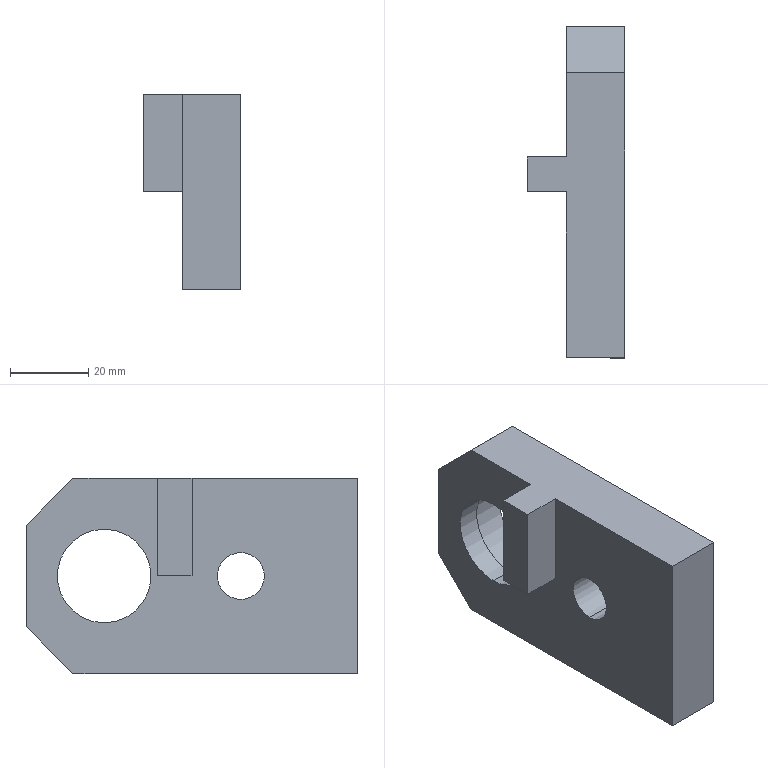Component | SolidWorks | BracketThree-1 | 1 solid | 19 faces | box 25 x 85 x 50 mm | volume 54632 mm3 | plane 13 | cylinder 6 | commonest cylinder face diameters 24 x2 26 x2 12 x2
build123d program:
from build123d import *

# Parameters (mm, degrees)
SKETCH1_R           = 6
BOSS_EXTRUDE1_DEPTH = 15
SKETCH2_R           = 13
CUT_EXTRUDE1_DEPTH  = 9
CUT_EXTRUDE2_REACH  = 52.122
SKETCH3_R           = 12
SKETCH4_W           = 25
SKETCH4_H           = 8.926
BOSS_EXTRUDE2_DEPTH = 10


with BuildPart() as part:
    # Sketch1 → Boss-Extrude1 (new body)
    with BuildSketch(Plane.XY):
        Polygon((-25, 30.5), (-13, 42.5), (13, 42.5), (25, 30.5), (25, -42.5), (-25, -42.5), align=None)
        with Locations((0, -12.5)):
            Circle(SKETCH1_R, mode=Mode.SUBTRACT)
    extrude(amount=BOSS_EXTRUDE1_DEPTH)

    # Sketch2 → Cut-Extrude1 (cut)
    with BuildSketch(Plane.XY.offset(15)):
        with Locations((0, 22.5)):
            Circle(SKETCH2_R)
    extrude(amount=-CUT_EXTRUDE1_DEPTH, mode=Mode.SUBTRACT)

    # Sketch3 → Cut-Extrude2 (cut, up to next)
    with BuildSketch(Plane.XY.offset(6), mode=Mode.PRIVATE) as cut_extrude2_sk1:
        with Locations((0, 22.5)):
            Circle(SKETCH3_R)
    cut_extrude2_tool1 = extrude(cut_extrude2_sk1.sketch, amount=-CUT_EXTRUDE2_REACH, mode=Mode.PRIVATE) & part.part
    add(cut_extrude2_tool1.solids().sort_by_distance((0, 22.5, 6))[0], mode=Mode.SUBTRACT)

    # Sketch4 → Boss-Extrude2 (add)
    with BuildSketch(Plane(origin=(0, 0, 0), x_dir=(-1, 0, 0), z_dir=(0, 0, -1))):
        with Locations((12.5, 4.463)):
            Rectangle(SKETCH4_W, SKETCH4_H)
    extrude(amount=BOSS_EXTRUDE2_DEPTH)


solid = part.part

# Placed as in the assembly
solid = solid.moved(Location((78.546, 54.5, 438.671), (0, 90, 0)))
STEP:
#1=CARTESIAN_POINT('',(3.092,3.031,16.798));
#2=VERTEX_POINT('',#1);
#3=CARTESIAN_POINT('',(3.092,3.031,17.743));
#4=VERTEX_POINT('',#3);
#5=CARTESIAN_POINT('',(3.092,3.031,17.271));
#6=DIRECTION('',(-1.,-0.,0.));
#7=DIRECTION('',(-0.,0.,-1.));
#8=AXIS2_PLACEMENT_3D('',#5,#6,#7);
#9=CIRCLE('',#8,0.4724);
#10=EDGE_CURVE('',#2,#4,#9,.T.);
#11=ORIENTED_EDGE('',*,*,#10,.T.);
#12=CARTESIAN_POINT('',(3.329,3.031,17.743));
#13=VERTEX_POINT('',#12);
#14=CARTESIAN_POINT('',(3.092,3.031,17.743));
#15=DIRECTION('',(1.,0.,-0.));
#16=VECTOR('',#15,39.37);
#17=LINE('',#14,#16);
#18=EDGE_CURVE('',#4,#13,#17,.T.);
#19=ORIENTED_EDGE('',*,*,#18,.T.);
#20=CARTESIAN_POINT('',(3.329,3.031,16.798));
#21=VERTEX_POINT('',#20);
#22=CARTESIAN_POINT('',(3.329,3.031,17.271));
#23=DIRECTION('',(1.,0.,-0.));
#24=DIRECTION('',(-0.,0.,-1.));
#25=AXIS2_PLACEMENT_3D('',#22,#23,#24);
#26=CIRCLE('',#25,0.4724);
#27=EDGE_CURVE('',#13,#21,#26,.T.);
#28=ORIENTED_EDGE('',*,*,#27,.T.);
#29=CARTESIAN_POINT('',(3.092,3.031,16.798));
#30=DIRECTION('',(1.,0.,-0.));
#31=VECTOR('',#30,39.37);
#32=LINE('',#29,#31);
#33=EDGE_CURVE('',#2,#21,#32,.T.);
#34=ORIENTED_EDGE('',*,*,#33,.F.);
#35=EDGE_LOOP('',(#11,#19,#28,#34));
#36=FACE_OUTER_BOUND('',#35,.T.);
#37=CARTESIAN_POINT('',(3.092,3.031,17.271));
#38=DIRECTION('',(1.,0.,-0.));
#39=DIRECTION('',(-0.,0.,-1.));
#40=AXIS2_PLACEMENT_3D('',#37,#38,#39);
#41=CYLINDRICAL_SURFACE('',#40,0.4724);
#42=ADVANCED_FACE('',(#36),#41,.F.);
#43=CARTESIAN_POINT('',(3.329,3.031,17.782));
#44=VERTEX_POINT('',#43);
#45=CARTESIAN_POINT('',(3.329,3.031,16.759));
#46=VERTEX_POINT('',#45);
#47=CARTESIAN_POINT('',(3.329,3.031,17.271));
#48=DIRECTION('',(1.,0.,-0.));
#49=DIRECTION('',(-0.,0.,-1.));
#50=AXIS2_PLACEMENT_3D('',#47,#48,#49);
#51=CIRCLE('',#50,0.5118);
#52=EDGE_CURVE('',#44,#46,#51,.T.);
#53=ORIENTED_EDGE('',*,*,#52,.F.);
#54=CARTESIAN_POINT('',(3.683,3.031,17.782));
#55=VERTEX_POINT('',#54);
#56=CARTESIAN_POINT('',(3.329,3.031,17.782));
#57=DIRECTION('',(1.,0.,-0.));
#58=VECTOR('',#57,39.37);
#59=LINE('',#56,#58);
#60=EDGE_CURVE('',#44,#55,#59,.T.);
#61=ORIENTED_EDGE('',*,*,#60,.T.);
#62=CARTESIAN_POINT('',(3.683,3.031,16.759));
#63=VERTEX_POINT('',#62);
#64=CARTESIAN_POINT('',(3.683,3.031,17.271));
#65=DIRECTION('',(1.,0.,-0.));
#66=DIRECTION('',(-0.,0.,-1.));
#67=AXIS2_PLACEMENT_3D('',#64,#65,#66);
#68=CIRCLE('',#67,0.5118);
#69=EDGE_CURVE('',#55,#63,#68,.T.);
#70=ORIENTED_EDGE('',*,*,#69,.T.);
#71=CARTESIAN_POINT('',(3.329,3.031,16.759));
#72=DIRECTION('',(1.,0.,-0.));
#73=VECTOR('',#72,39.37);
#74=LINE('',#71,#73);
#75=EDGE_CURVE('',#46,#63,#74,.T.);
#76=ORIENTED_EDGE('',*,*,#75,.F.);
#77=EDGE_LOOP('',(#53,#61,#70,#76));
#78=FACE_OUTER_BOUND('',#77,.T.);
#79=CARTESIAN_POINT('',(3.329,3.031,17.271));
#80=DIRECTION('',(1.,0.,-0.));
#81=DIRECTION('',(-0.,0.,-1.));
#82=AXIS2_PLACEMENT_3D('',#79,#80,#81);
#83=CYLINDRICAL_SURFACE('',#82,0.5118);
#84=ADVANCED_FACE('',(#78),#83,.F.);
#85=CARTESIAN_POINT('',(3.683,1.654,17.507));
#86=VERTEX_POINT('',#85);
#87=CARTESIAN_POINT('',(3.683,1.654,17.034));
#88=VERTEX_POINT('',#87);
#89=CARTESIAN_POINT('',(3.683,1.654,17.271));
#90=DIRECTION('',(1.,0.,-0.));
#91=DIRECTION('',(-0.,0.,-1.));
#92=AXIS2_PLACEMENT_3D('',#89,#90,#91);
#93=CIRCLE('',#92,0.2362);
#94=EDGE_CURVE('',#86,#88,#93,.T.);
#95=ORIENTED_EDGE('',*,*,#94,.T.);
#96=CARTESIAN_POINT('',(3.092,1.654,17.034));
#97=VERTEX_POINT('',#96);
#98=CARTESIAN_POINT('',(3.683,1.654,17.034));
#99=DIRECTION('',(-1.,-0.,0.));
#100=VECTOR('',#99,39.37);
#101=LINE('',#98,#100);
#102=EDGE_CURVE('',#88,#97,#101,.T.);
#103=ORIENTED_EDGE('',*,*,#102,.T.);
#104=CARTESIAN_POINT('',(3.092,1.654,17.507));
#105=VERTEX_POINT('',#104);
#106=CARTESIAN_POINT('',(3.092,1.654,17.271));
#107=DIRECTION('',(1.,0.,-0.));
#108=DIRECTION('',(-0.,0.,-1.));
#109=AXIS2_PLACEMENT_3D('',#106,#107,#108);
#110=CIRCLE('',#109,0.2362);
#111=EDGE_CURVE('',#105,#97,#110,.T.);
#112=ORIENTED_EDGE('',*,*,#111,.F.);
#113=CARTESIAN_POINT('',(3.683,1.654,17.507));
#114=DIRECTION('',(-1.,-0.,0.));
#115=VECTOR('',#114,39.37);
#116=LINE('',#113,#115);
#117=EDGE_CURVE('',#86,#105,#116,.T.);
#118=ORIENTED_EDGE('',*,*,#117,.F.);
#119=EDGE_LOOP('',(#95,#103,#112,#118));
#120=FACE_OUTER_BOUND('',#119,.T.);
#121=CARTESIAN_POINT('',(3.683,1.654,17.271));
#122=DIRECTION('',(-1.,-0.,0.));
#123=DIRECTION('',(0.,0.,1.));
#124=AXIS2_PLACEMENT_3D('',#121,#122,#123);
#125=CYLINDRICAL_SURFACE('',#124,0.2362);
#126=ADVANCED_FACE('',(#120),#125,.F.);
#127=ORIENTED_EDGE('',*,*,#111,.T.);
#128=CARTESIAN_POINT('',(3.092,1.654,17.271));
#129=DIRECTION('',(1.,0.,-0.));
#130=DIRECTION('',(-0.,0.,-1.));
#131=AXIS2_PLACEMENT_3D('',#128,#129,#130);
#132=CIRCLE('',#131,0.2362);
#133=EDGE_CURVE('',#97,#105,#132,.T.);
#134=ORIENTED_EDGE('',*,*,#133,.T.);
#135=EDGE_LOOP('',(#127,#134));
#136=FACE_BOUND('',#135,.T.);
#137=ORIENTED_EDGE('',*,*,#10,.F.);
#138=CARTESIAN_POINT('',(3.092,3.031,17.271));
#139=DIRECTION('',(-1.,-0.,0.));
#140=DIRECTION('',(-0.,0.,-1.));
#141=AXIS2_PLACEMENT_3D('',#138,#139,#140);
#142=CIRCLE('',#141,0.4724);
#143=EDGE_CURVE('',#4,#2,#142,.T.);
#144=ORIENTED_EDGE('',*,*,#143,.F.);
#145=EDGE_LOOP('',(#137,#144));
#146=FACE_BOUND('',#145,.T.);
#147=CARTESIAN_POINT('',(3.092,2.497,18.255));
#148=VERTEX_POINT('',#147);
#149=CARTESIAN_POINT('',(3.092,2.497,17.271));
#150=VERTEX_POINT('',#149);
#151=CARTESIAN_POINT('',(3.092,2.497,17.271));
#152=DIRECTION('',(-0.,-0.,-1.));
#153=VECTOR('',#152,39.37);
#154=LINE('',#151,#153);
#155=EDGE_CURVE('',#148,#150,#154,.T.);
#156=ORIENTED_EDGE('',*,*,#155,.F.);
#157=CARTESIAN_POINT('',(3.092,3.346,18.255));
#158=VERTEX_POINT('',#157);
#159=CARTESIAN_POINT('',(3.092,3.346,18.255));
#160=DIRECTION('',(0.,-1.,-0.));
#161=VECTOR('',#160,39.37);
#162=LINE('',#159,#161);
#163=EDGE_CURVE('',#158,#148,#162,.T.);
#164=ORIENTED_EDGE('',*,*,#163,.F.);
#165=CARTESIAN_POINT('',(3.092,3.819,17.782));
#166=VERTEX_POINT('',#165);
#167=CARTESIAN_POINT('',(3.092,3.346,18.255));
#168=DIRECTION('',(0.,-0.7071,0.7071));
#169=VECTOR('',#168,39.37);
#170=LINE('',#167,#169);
#171=EDGE_CURVE('',#166,#158,#170,.T.);
#172=ORIENTED_EDGE('',*,*,#171,.F.);
#173=CARTESIAN_POINT('',(3.092,3.819,16.759));
#174=VERTEX_POINT('',#173);
#175=CARTESIAN_POINT('',(3.092,3.819,17.782));
#176=DIRECTION('',(0.,0.,1.));
#177=VECTOR('',#176,39.37);
#178=LINE('',#175,#177);
#179=EDGE_CURVE('',#174,#166,#178,.T.);
#180=ORIENTED_EDGE('',*,*,#179,.F.);
#181=CARTESIAN_POINT('',(3.092,3.346,16.286));
#182=VERTEX_POINT('',#181);
#183=CARTESIAN_POINT('',(3.092,3.819,16.759));
#184=DIRECTION('',(0.,0.7071,0.7071));
#185=VECTOR('',#184,39.37);
#186=LINE('',#183,#185);
#187=EDGE_CURVE('',#182,#174,#186,.T.);
#188=ORIENTED_EDGE('',*,*,#187,.F.);
#189=CARTESIAN_POINT('',(3.092,0.4724,16.286));
#190=VERTEX_POINT('',#189);
#191=CARTESIAN_POINT('',(3.092,3.346,16.286));
#192=DIRECTION('',(-0.,1.,-0.));
#193=VECTOR('',#192,39.37);
#194=LINE('',#191,#193);
#195=EDGE_CURVE('',#190,#182,#194,.T.);
#196=ORIENTED_EDGE('',*,*,#195,.F.);
#197=CARTESIAN_POINT('',(3.092,0.4724,18.255));
#198=VERTEX_POINT('',#197);
#199=CARTESIAN_POINT('',(3.092,0.4724,18.255));
#200=DIRECTION('',(-0.,-0.,-1.));
#201=VECTOR('',#200,39.37);
#202=LINE('',#199,#201);
#203=EDGE_CURVE('',#198,#190,#202,.T.);
#204=ORIENTED_EDGE('',*,*,#203,.F.);
#205=CARTESIAN_POINT('',(3.092,2.146,18.255));
#206=VERTEX_POINT('',#205);
#207=CARTESIAN_POINT('',(3.092,3.346,18.255));
#208=DIRECTION('',(0.,-1.,-0.));
#209=VECTOR('',#208,39.37);
#210=LINE('',#207,#209);
#211=EDGE_CURVE('',#206,#198,#210,.T.);
#212=ORIENTED_EDGE('',*,*,#211,.F.);
#213=CARTESIAN_POINT('',(3.092,2.146,17.271));
#214=VERTEX_POINT('',#213);
#215=CARTESIAN_POINT('',(3.092,2.146,17.271));
#216=DIRECTION('',(0.,0.,1.));
#217=VECTOR('',#216,39.37);
#218=LINE('',#215,#217);
#219=EDGE_CURVE('',#214,#206,#218,.T.);
#220=ORIENTED_EDGE('',*,*,#219,.F.);
#221=CARTESIAN_POINT('',(3.092,2.146,17.271));
#222=DIRECTION('',(0.,-1.,0.));
#223=VECTOR('',#222,39.37);
#224=LINE('',#221,#223);
#225=EDGE_CURVE('',#150,#214,#224,.T.);
#226=ORIENTED_EDGE('',*,*,#225,.F.);
#227=EDGE_LOOP('',(#156,#164,#172,#180,#188,#196,#204,#212,#220,#226));
#228=FACE_OUTER_BOUND('',#227,.T.);
#229=CARTESIAN_POINT('',(3.092,2.146,17.271));
#230=DIRECTION('',(1.,0.,-0.));
#231=DIRECTION('',(-0.,-0.,-1.));
#232=AXIS2_PLACEMENT_3D('',#229,#230,#231);
#233=PLANE('',#232);
#234=ADVANCED_FACE('',(#136,#146,#228),#233,.F.);
#235=CARTESIAN_POINT('',(3.683,3.031,17.271));
#236=DIRECTION('',(1.,0.,-0.));
#237=DIRECTION('',(-0.,0.,-1.));
#238=AXIS2_PLACEMENT_3D('',#235,#236,#237);
#239=CIRCLE('',#238,0.5118);
#240=EDGE_CURVE('',#63,#55,#239,.T.);
#241=ORIENTED_EDGE('',*,*,#240,.F.);
#242=ORIENTED_EDGE('',*,*,#69,.F.);
#243=EDGE_LOOP('',(#241,#242));
#244=FACE_BOUND('',#243,.T.);
#245=CARTESIAN_POINT('',(3.683,0.4724,16.286));
#246=VERTEX_POINT('',#245);
#247=CARTESIAN_POINT('',(3.683,3.346,16.286));
#248=VERTEX_POINT('',#247);
#249=CARTESIAN_POINT('',(3.683,3.346,16.286));
#250=DIRECTION('',(-0.,1.,-0.));
#251=VECTOR('',#250,39.37);
#252=LINE('',#249,#251);
#253=EDGE_CURVE('',#246,#248,#252,.T.);
#254=ORIENTED_EDGE('',*,*,#253,.T.);
#255=CARTESIAN_POINT('',(3.683,3.819,16.759));
#256=VERTEX_POINT('',#255);
#257=CARTESIAN_POINT('',(3.683,3.819,16.759));
#258=DIRECTION('',(0.,0.7071,0.7071));
#259=VECTOR('',#258,39.37);
#260=LINE('',#257,#259);
#261=EDGE_CURVE('',#248,#256,#260,.T.);
#262=ORIENTED_EDGE('',*,*,#261,.T.);
#263=CARTESIAN_POINT('',(3.683,3.819,17.782));
#264=VERTEX_POINT('',#263);
#265=CARTESIAN_POINT('',(3.683,3.819,17.782));
#266=DIRECTION('',(0.,0.,1.));
#267=VECTOR('',#266,39.37);
#268=LINE('',#265,#267);
#269=EDGE_CURVE('',#256,#264,#268,.T.);
#270=ORIENTED_EDGE('',*,*,#269,.T.);
#271=CARTESIAN_POINT('',(3.683,3.346,18.255));
#272=VERTEX_POINT('',#271);
#273=CARTESIAN_POINT('',(3.683,3.346,18.255));
#274=DIRECTION('',(0.,-0.7071,0.7071));
#275=VECTOR('',#274,39.37);
#276=LINE('',#273,#275);
#277=EDGE_CURVE('',#264,#272,#276,.T.);
#278=ORIENTED_EDGE('',*,*,#277,.T.);
#279=CARTESIAN_POINT('',(3.683,0.4724,18.255));
#280=VERTEX_POINT('',#279);
#281=CARTESIAN_POINT('',(3.683,3.346,18.255));
#282=DIRECTION('',(0.,-1.,-0.));
#283=VECTOR('',#282,39.37);
#284=LINE('',#281,#283);
#285=EDGE_CURVE('',#272,#280,#284,.T.);
#286=ORIENTED_EDGE('',*,*,#285,.T.);
#287=CARTESIAN_POINT('',(3.683,0.4724,18.255));
#288=DIRECTION('',(-0.,-0.,-1.));
#289=VECTOR('',#288,39.37);
#290=LINE('',#287,#289);
#291=EDGE_CURVE('',#280,#246,#290,.T.);
#292=ORIENTED_EDGE('',*,*,#291,.T.);
#293=EDGE_LOOP('',(#254,#262,#270,#278,#286,#292));
#294=FACE_OUTER_BOUND('',#293,.T.);
#295=ORIENTED_EDGE('',*,*,#94,.F.);
#296=CARTESIAN_POINT('',(3.683,1.654,17.271));
#297=DIRECTION('',(1.,0.,-0.));
#298=DIRECTION('',(-0.,0.,-1.));
#299=AXIS2_PLACEMENT_3D('',#296,#297,#298);
#300=CIRCLE('',#299,0.2362);
#301=EDGE_CURVE('',#88,#86,#300,.T.);
#302=ORIENTED_EDGE('',*,*,#301,.F.);
#303=EDGE_LOOP('',(#295,#302));
#304=FACE_BOUND('',#303,.T.);
#305=CARTESIAN_POINT('',(3.683,2.146,17.271));
#306=DIRECTION('',(1.,0.,-0.));
#307=DIRECTION('',(-0.,-0.,-1.));
#308=AXIS2_PLACEMENT_3D('',#305,#306,#307);
#309=PLANE('',#308);
#310=ADVANCED_FACE('',(#244,#294,#304),#309,.T.);
#311=ORIENTED_EDGE('',*,*,#195,.T.);
#312=CARTESIAN_POINT('',(3.683,3.346,16.286));
#313=DIRECTION('',(-1.,-0.,0.));
#314=VECTOR('',#313,39.37);
#315=LINE('',#312,#314);
#316=EDGE_CURVE('',#248,#182,#315,.T.);
#317=ORIENTED_EDGE('',*,*,#316,.F.);
#318=ORIENTED_EDGE('',*,*,#253,.F.);
#319=CARTESIAN_POINT('',(3.683,0.4724,16.286));
#320=DIRECTION('',(-1.,-0.,0.));
#321=VECTOR('',#320,39.37);
#322=LINE('',#319,#321);
#323=EDGE_CURVE('',#246,#190,#322,.T.);
#324=ORIENTED_EDGE('',*,*,#323,.T.);
#325=EDGE_LOOP('',(#311,#317,#318,#324));
#326=FACE_OUTER_BOUND('',#325,.T.);
#327=CARTESIAN_POINT('',(3.683,3.346,16.286));
#328=DIRECTION('',(0.,0.,1.));
#329=DIRECTION('',(0.,-1.,0.));
#330=AXIS2_PLACEMENT_3D('',#327,#328,#329);
#331=PLANE('',#330);
#332=ADVANCED_FACE('',(#326),#331,.F.);
#333=ORIENTED_EDGE('',*,*,#187,.T.);
#334=CARTESIAN_POINT('',(3.683,3.819,16.759));
#335=DIRECTION('',(-1.,-0.,0.));
#336=VECTOR('',#335,39.37);
#337=LINE('',#334,#336);
#338=EDGE_CURVE('',#256,#174,#337,.T.);
#339=ORIENTED_EDGE('',*,*,#338,.F.);
#340=ORIENTED_EDGE('',*,*,#261,.F.);
#341=ORIENTED_EDGE('',*,*,#316,.T.);
#342=EDGE_LOOP('',(#333,#339,#340,#341));
#343=FACE_OUTER_BOUND('',#342,.T.);
#344=CARTESIAN_POINT('',(3.683,3.819,16.759));
#345=DIRECTION('',(0.,-0.7071,0.7071));
#346=DIRECTION('',(-0.,-0.7071,-0.7071));
#347=AXIS2_PLACEMENT_3D('',#344,#345,#346);
#348=PLANE('',#347);
#349=ADVANCED_FACE('',(#343),#348,.F.);
#350=ORIENTED_EDGE('',*,*,#179,.T.);
#351=CARTESIAN_POINT('',(3.683,3.819,17.782));
#352=DIRECTION('',(-1.,-0.,0.));
#353=VECTOR('',#352,39.37);
#354=LINE('',#351,#353);
#355=EDGE_CURVE('',#264,#166,#354,.T.);
#356=ORIENTED_EDGE('',*,*,#355,.F.);
#357=ORIENTED_EDGE('',*,*,#269,.F.);
#358=ORIENTED_EDGE('',*,*,#338,.T.);
#359=EDGE_LOOP('',(#350,#356,#357,#358));
#360=FACE_OUTER_BOUND('',#359,.T.);
#361=CARTESIAN_POINT('',(3.683,3.819,17.782));
#362=DIRECTION('',(0.,-1.,0.));
#363=DIRECTION('',(-1.,-0.,0.));
#364=AXIS2_PLACEMENT_3D('',#361,#362,#363);
#365=PLANE('',#364);
#366=ADVANCED_FACE('',(#360),#365,.F.);
#367=ORIENTED_EDGE('',*,*,#171,.T.);
#368=CARTESIAN_POINT('',(3.683,3.346,18.255));
#369=DIRECTION('',(-1.,-0.,0.));
#370=VECTOR('',#369,39.37);
#371=LINE('',#368,#370);
#372=EDGE_CURVE('',#272,#158,#371,.T.);
#373=ORIENTED_EDGE('',*,*,#372,.F.);
#374=ORIENTED_EDGE('',*,*,#277,.F.);
#375=ORIENTED_EDGE('',*,*,#355,.T.);
#376=EDGE_LOOP('',(#367,#373,#374,#375));
#377=FACE_OUTER_BOUND('',#376,.T.);
#378=CARTESIAN_POINT('',(3.683,3.346,18.255));
#379=DIRECTION('',(-0.,-0.7071,-0.7071));
#380=DIRECTION('',(-0.,0.7071,-0.7071));
#381=AXIS2_PLACEMENT_3D('',#378,#379,#380);
#382=PLANE('',#381);
#383=ADVANCED_FACE('',(#377),#382,.F.);
#384=ORIENTED_EDGE('',*,*,#163,.T.);
#385=CARTESIAN_POINT('',(2.699,2.497,18.255));
#386=VERTEX_POINT('',#385);
#387=CARTESIAN_POINT('',(2.699,2.497,18.255));
#388=DIRECTION('',(1.,0.,-0.));
#389=VECTOR('',#388,39.37);
#390=LINE('',#387,#389);
#391=EDGE_CURVE('',#386,#148,#390,.T.);
#392=ORIENTED_EDGE('',*,*,#391,.F.);
#393=CARTESIAN_POINT('',(2.699,2.146,18.255));
#394=VERTEX_POINT('',#393);
#395=CARTESIAN_POINT('',(2.699,2.146,18.255));
#396=DIRECTION('',(-0.,1.,-0.));
#397=VECTOR('',#396,39.37);
#398=LINE('',#395,#397);
#399=EDGE_CURVE('',#394,#386,#398,.T.);
#400=ORIENTED_EDGE('',*,*,#399,.F.);
#401=CARTESIAN_POINT('',(2.699,2.146,18.255));
#402=DIRECTION('',(1.,0.,-0.));
#403=VECTOR('',#402,39.37);
#404=LINE('',#401,#403);
#405=EDGE_CURVE('',#394,#206,#404,.T.);
#406=ORIENTED_EDGE('',*,*,#405,.T.);
#407=ORIENTED_EDGE('',*,*,#211,.T.);
#408=CARTESIAN_POINT('',(3.683,0.4724,18.255));
#409=DIRECTION('',(-1.,-0.,0.));
#410=VECTOR('',#409,39.37);
#411=LINE('',#408,#410);
#412=EDGE_CURVE('',#280,#198,#411,.T.);
#413=ORIENTED_EDGE('',*,*,#412,.F.);
#414=ORIENTED_EDGE('',*,*,#285,.F.);
#415=ORIENTED_EDGE('',*,*,#372,.T.);
#416=EDGE_LOOP('',(#384,#392,#400,#406,#407,#413,#414,#415));
#417=FACE_OUTER_BOUND('',#416,.T.);
#418=CARTESIAN_POINT('',(3.683,3.346,18.255));
#419=DIRECTION('',(-0.,0.,-1.));
#420=DIRECTION('',(-0.,1.,0.));
#421=AXIS2_PLACEMENT_3D('',#418,#419,#420);
#422=PLANE('',#421);
#423=ADVANCED_FACE('',(#417),#422,.F.);
#424=ORIENTED_EDGE('',*,*,#203,.T.);
#425=ORIENTED_EDGE('',*,*,#323,.F.);
#426=ORIENTED_EDGE('',*,*,#291,.F.);
#427=ORIENTED_EDGE('',*,*,#412,.T.);
#428=EDGE_LOOP('',(#424,#425,#426,#427));
#429=FACE_OUTER_BOUND('',#428,.T.);
#430=CARTESIAN_POINT('',(3.683,0.4724,18.255));
#431=DIRECTION('',(-0.,1.,-0.));
#432=DIRECTION('',(1.,0.,-0.));
#433=AXIS2_PLACEMENT_3D('',#430,#431,#432);
#434=PLANE('',#433);
#435=ADVANCED_FACE('',(#429),#434,.F.);
#436=ORIENTED_EDGE('',*,*,#102,.F.);
#437=ORIENTED_EDGE('',*,*,#301,.T.);
#438=ORIENTED_EDGE('',*,*,#117,.T.);
#439=ORIENTED_EDGE('',*,*,#133,.F.);
#440=EDGE_LOOP('',(#436,#437,#438,#439));
#441=FACE_OUTER_BOUND('',#440,.T.);
#442=CARTESIAN_POINT('',(3.683,1.654,17.271));
#443=DIRECTION('',(-1.,-0.,0.));
#444=DIRECTION('',(0.,0.,1.));
#445=AXIS2_PLACEMENT_3D('',#442,#443,#444);
#446=CYLINDRICAL_SURFACE('',#445,0.2362);
#447=ADVANCED_FACE('',(#441),#446,.F.);
#448=ORIENTED_EDGE('',*,*,#60,.F.);
#449=CARTESIAN_POINT('',(3.329,3.031,17.271));
#450=DIRECTION('',(1.,0.,-0.));
#451=DIRECTION('',(-0.,0.,-1.));
#452=AXIS2_PLACEMENT_3D('',#449,#450,#451);
#453=CIRCLE('',#452,0.5118);
#454=EDGE_CURVE('',#46,#44,#453,.T.);
#455=ORIENTED_EDGE('',*,*,#454,.F.);
#456=ORIENTED_EDGE('',*,*,#75,.T.);
#457=ORIENTED_EDGE('',*,*,#240,.T.);
#458=EDGE_LOOP('',(#448,#455,#456,#457));
#459=FACE_OUTER_BOUND('',#458,.T.);
#460=CARTESIAN_POINT('',(3.329,3.031,17.271));
#461=DIRECTION('',(1.,0.,-0.));
#462=DIRECTION('',(-0.,0.,-1.));
#463=AXIS2_PLACEMENT_3D('',#460,#461,#462);
#464=CYLINDRICAL_SURFACE('',#463,0.5118);
#465=ADVANCED_FACE('',(#459),#464,.F.);
#466=CARTESIAN_POINT('',(3.329,3.031,17.271));
#467=DIRECTION('',(1.,0.,-0.));
#468=DIRECTION('',(-0.,0.,-1.));
#469=AXIS2_PLACEMENT_3D('',#466,#467,#468);
#470=CIRCLE('',#469,0.4724);
#471=EDGE_CURVE('',#21,#13,#470,.T.);
#472=ORIENTED_EDGE('',*,*,#471,.F.);
#473=ORIENTED_EDGE('',*,*,#27,.F.);
#474=EDGE_LOOP('',(#472,#473));
#475=FACE_BOUND('',#474,.T.);
#476=ORIENTED_EDGE('',*,*,#454,.T.);
#477=ORIENTED_EDGE('',*,*,#52,.T.);
#478=EDGE_LOOP('',(#476,#477));
#479=FACE_OUTER_BOUND('',#478,.T.);
#480=CARTESIAN_POINT('',(3.329,3.031,17.271));
#481=DIRECTION('',(1.,0.,-0.));
#482=DIRECTION('',(-0.,-0.,-1.));
#483=AXIS2_PLACEMENT_3D('',#480,#481,#482);
#484=PLANE('',#483);
#485=ADVANCED_FACE('',(#475,#479),#484,.T.);
#486=ORIENTED_EDGE('',*,*,#18,.F.);
#487=ORIENTED_EDGE('',*,*,#143,.T.);
#488=ORIENTED_EDGE('',*,*,#33,.T.);
#489=ORIENTED_EDGE('',*,*,#471,.T.);
#490=EDGE_LOOP('',(#486,#487,#488,#489));
#491=FACE_OUTER_BOUND('',#490,.T.);
#492=CARTESIAN_POINT('',(3.092,3.031,17.271));
#493=DIRECTION('',(1.,0.,-0.));
#494=DIRECTION('',(-0.,0.,-1.));
#495=AXIS2_PLACEMENT_3D('',#492,#493,#494);
#496=CYLINDRICAL_SURFACE('',#495,0.4724);
#497=ADVANCED_FACE('',(#491),#496,.F.);
#498=ORIENTED_EDGE('',*,*,#225,.T.);
#499=CARTESIAN_POINT('',(2.699,2.146,17.271));
#500=VERTEX_POINT('',#499);
#501=CARTESIAN_POINT('',(2.699,2.146,17.271));
#502=DIRECTION('',(1.,0.,-0.));
#503=VECTOR('',#502,39.37);
#504=LINE('',#501,#503);
#505=EDGE_CURVE('',#500,#214,#504,.T.);
#506=ORIENTED_EDGE('',*,*,#505,.F.);
#507=CARTESIAN_POINT('',(2.699,2.497,17.271));
#508=VERTEX_POINT('',#507);
#509=CARTESIAN_POINT('',(2.699,2.146,17.271));
#510=DIRECTION('',(0.,-1.,0.));
#511=VECTOR('',#510,39.37);
#512=LINE('',#509,#511);
#513=EDGE_CURVE('',#508,#500,#512,.T.);
#514=ORIENTED_EDGE('',*,*,#513,.F.);
#515=CARTESIAN_POINT('',(2.699,2.497,17.271));
#516=DIRECTION('',(1.,0.,-0.));
#517=VECTOR('',#516,39.37);
#518=LINE('',#515,#517);
#519=EDGE_CURVE('',#508,#150,#518,.T.);
#520=ORIENTED_EDGE('',*,*,#519,.T.);
#521=EDGE_LOOP('',(#498,#506,#514,#520));
#522=FACE_OUTER_BOUND('',#521,.T.);
#523=CARTESIAN_POINT('',(2.699,2.146,17.271));
#524=DIRECTION('',(0.,0.,1.));
#525=DIRECTION('',(1.,0.,-0.));
#526=AXIS2_PLACEMENT_3D('',#523,#524,#525);
#527=PLANE('',#526);
#528=ADVANCED_FACE('',(#522),#527,.F.);
#529=ORIENTED_EDGE('',*,*,#219,.T.);
#530=ORIENTED_EDGE('',*,*,#405,.F.);
#531=CARTESIAN_POINT('',(2.699,2.146,17.271));
#532=DIRECTION('',(0.,0.,1.));
#533=VECTOR('',#532,39.37);
#534=LINE('',#531,#533);
#535=EDGE_CURVE('',#500,#394,#534,.T.);
#536=ORIENTED_EDGE('',*,*,#535,.F.);
#537=ORIENTED_EDGE('',*,*,#505,.T.);
#538=EDGE_LOOP('',(#529,#530,#536,#537));
#539=FACE_OUTER_BOUND('',#538,.T.);
#540=CARTESIAN_POINT('',(2.699,2.146,17.271));
#541=DIRECTION('',(-0.,1.,-0.));
#542=DIRECTION('',(1.,0.,-0.));
#543=AXIS2_PLACEMENT_3D('',#540,#541,#542);
#544=PLANE('',#543);
#545=ADVANCED_FACE('',(#539),#544,.F.);
#546=ORIENTED_EDGE('',*,*,#155,.T.);
#547=ORIENTED_EDGE('',*,*,#519,.F.);
#548=CARTESIAN_POINT('',(2.699,2.497,17.271));
#549=DIRECTION('',(-0.,-0.,-1.));
#550=VECTOR('',#549,39.37);
#551=LINE('',#548,#550);
#552=EDGE_CURVE('',#386,#508,#551,.T.);
#553=ORIENTED_EDGE('',*,*,#552,.F.);
#554=ORIENTED_EDGE('',*,*,#391,.T.);
#555=EDGE_LOOP('',(#546,#547,#553,#554));
#556=FACE_OUTER_BOUND('',#555,.T.);
#557=CARTESIAN_POINT('',(2.699,2.497,17.271));
#558=DIRECTION('',(0.,-1.,0.));
#559=DIRECTION('',(-1.,-0.,0.));
#560=AXIS2_PLACEMENT_3D('',#557,#558,#559);
#561=PLANE('',#560);
#562=ADVANCED_FACE('',(#556),#561,.F.);
#563=ORIENTED_EDGE('',*,*,#513,.T.);
#564=ORIENTED_EDGE('',*,*,#535,.T.);
#565=ORIENTED_EDGE('',*,*,#399,.T.);
#566=ORIENTED_EDGE('',*,*,#552,.T.);
#567=EDGE_LOOP('',(#563,#564,#565,#566));
#568=FACE_OUTER_BOUND('',#567,.T.);
#569=CARTESIAN_POINT('',(2.699,2.146,17.271));
#570=DIRECTION('',(1.,0.,-0.));
#571=DIRECTION('',(-0.,-0.,-1.));
#572=AXIS2_PLACEMENT_3D('',#569,#570,#571);
#573=PLANE('',#572);
#574=ADVANCED_FACE('',(#568),#573,.F.);
#575=CLOSED_SHELL('',(#42,#84,#126,#234,#310,#332,#349,#366,#383,#423,#435,#447,#465,#485,#497,#528,#545,#562,#574));
#576=MANIFOLD_SOLID_BREP('',#575);
#577=CARTESIAN_POINT('',(0.,0.,0.));
#578=DIRECTION('',(0.,0.,1.));
#579=DIRECTION('',(1.,0.,0.));
#580=AXIS2_PLACEMENT_3D('',#577,#578,#579);
#581=(LENGTH_UNIT()NAMED_UNIT(*)SI_UNIT($,.METRE.));
#582=LENGTH_MEASURE_WITH_UNIT(LENGTH_MEASURE(0.0254),#581);
#583=DIMENSIONAL_EXPONENTS(1.,0.,0.,0.,0.,0.,0.);
#584=(CONVERSION_BASED_UNIT('',#582)LENGTH_UNIT()NAMED_UNIT(#583));
#585=UNCERTAINTY_MEASURE_WITH_UNIT(LENGTH_MEASURE(0.00001),#584,'','');
#586=(NAMED_UNIT(*)PLANE_ANGLE_UNIT()SI_UNIT($,.RADIAN.));
#587=(NAMED_UNIT(*)SI_UNIT($,.STERADIAN.)SOLID_ANGLE_UNIT());
#588=(GEOMETRIC_REPRESENTATION_CONTEXT(3)GLOBAL_UNCERTAINTY_ASSIGNED_CONTEXT((#585))GLOBAL_UNIT_ASSIGNED_CONTEXT((#584,#586,#587))REPRESENTATION_CONTEXT('',''));
#589=ADVANCED_BREP_SHAPE_REPRESENTATION('',(#576,#580),#588);
#590=COLOUR_RGB('',0.7922,0.8196,0.9333);
#591=FILL_AREA_STYLE_COLOUR('',#590);
#592=FILL_AREA_STYLE('',(#591));
#593=SURFACE_STYLE_FILL_AREA(#592);
#594=SURFACE_SIDE_STYLE('',(#593));
#595=SURFACE_STYLE_USAGE(.BOTH.,#594);
#596=PRESENTATION_STYLE_ASSIGNMENT((#595));
#597=STYLED_ITEM('',(#596),#576);
#598=PRESENTATION_LAYER_ASSIGNMENT('','',(#597));
#599=(LENGTH_UNIT()NAMED_UNIT(*)SI_UNIT($,.METRE.));
#600=LENGTH_MEASURE_WITH_UNIT(LENGTH_MEASURE(0.0254),#599);
#601=DIMENSIONAL_EXPONENTS(1.,0.,0.,0.,0.,0.,0.);
#602=(CONVERSION_BASED_UNIT('',#600)LENGTH_UNIT()NAMED_UNIT(#601));
#603=UNCERTAINTY_MEASURE_WITH_UNIT(LENGTH_MEASURE(0.00001),#602,'','');
#604=(NAMED_UNIT(*)PLANE_ANGLE_UNIT()SI_UNIT($,.RADIAN.));
#605=(NAMED_UNIT(*)SI_UNIT($,.STERADIAN.)SOLID_ANGLE_UNIT());
#606=(GEOMETRIC_REPRESENTATION_CONTEXT(3)GLOBAL_UNCERTAINTY_ASSIGNED_CONTEXT((#603))GLOBAL_UNIT_ASSIGNED_CONTEXT((#602,#604,#605))REPRESENTATION_CONTEXT('',''));
#607=MECHANICAL_DESIGN_GEOMETRIC_PRESENTATION_REPRESENTATION('',(#597),#606);